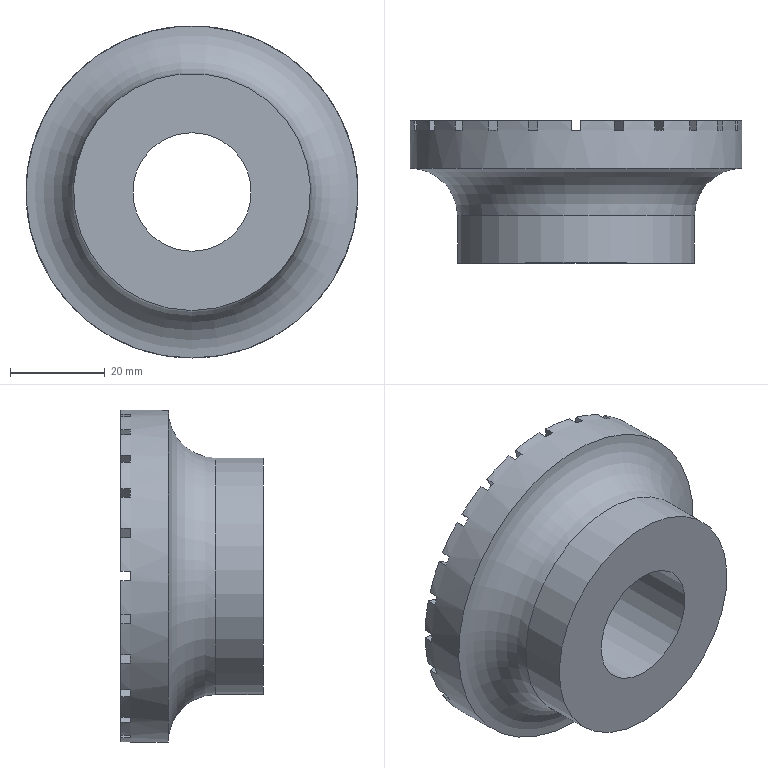Component | NX | TOP_PAD | 1 solid | 103 faces | volume 60055 mm3 | plane 98 | cylinder 4 | torus 1 | commonest cylinder face diameters 70 x1 50 x1 25 x1 35.5 x1